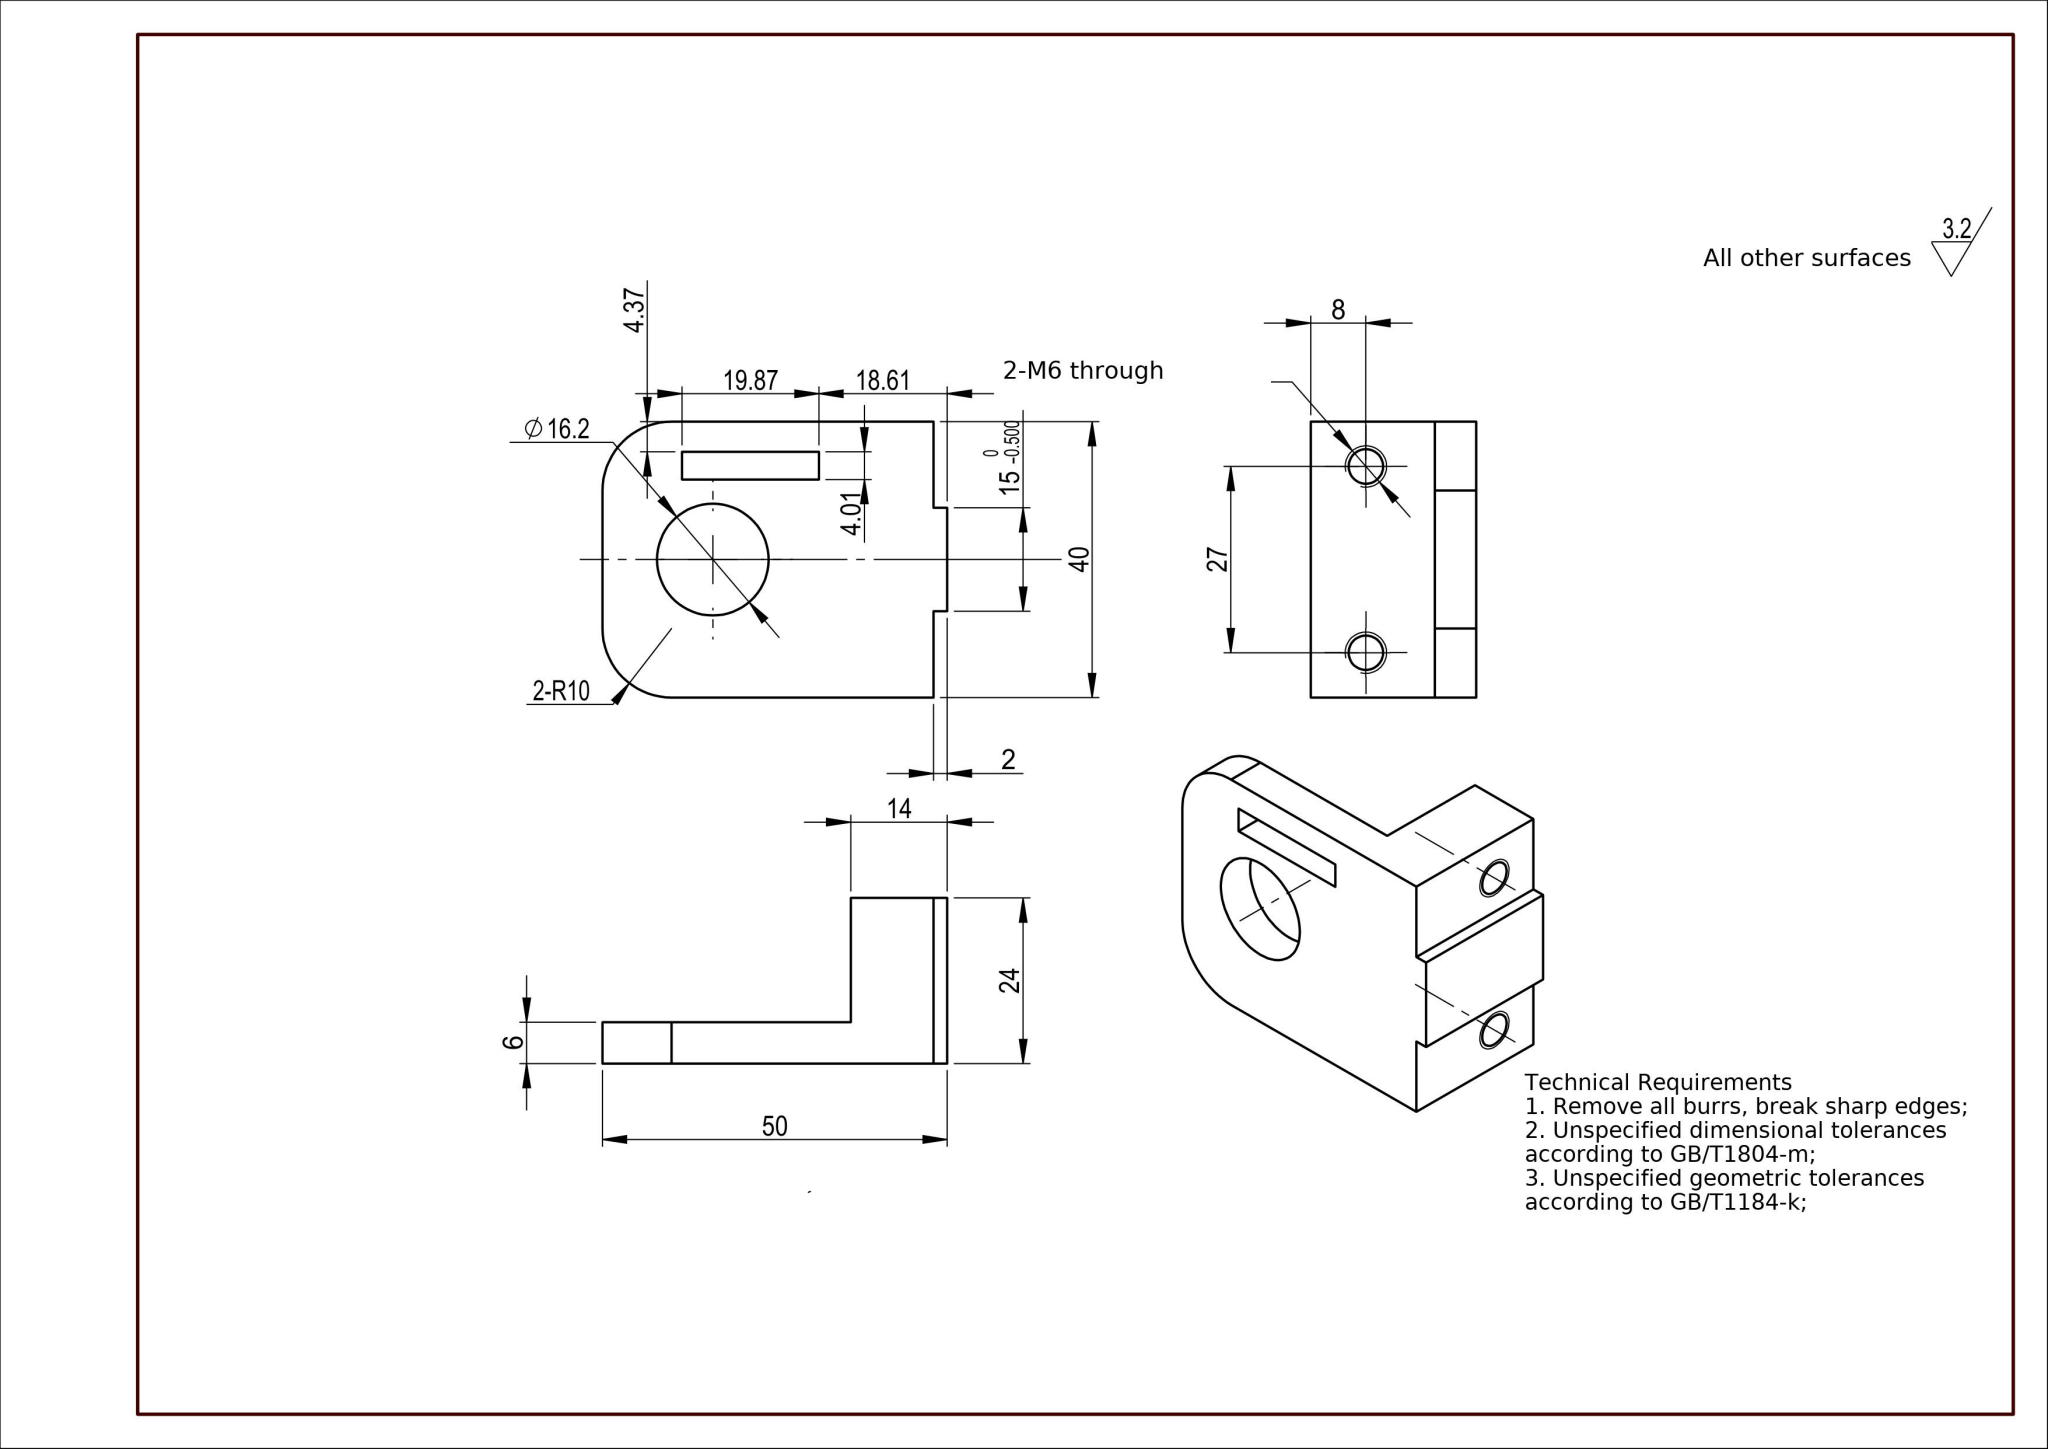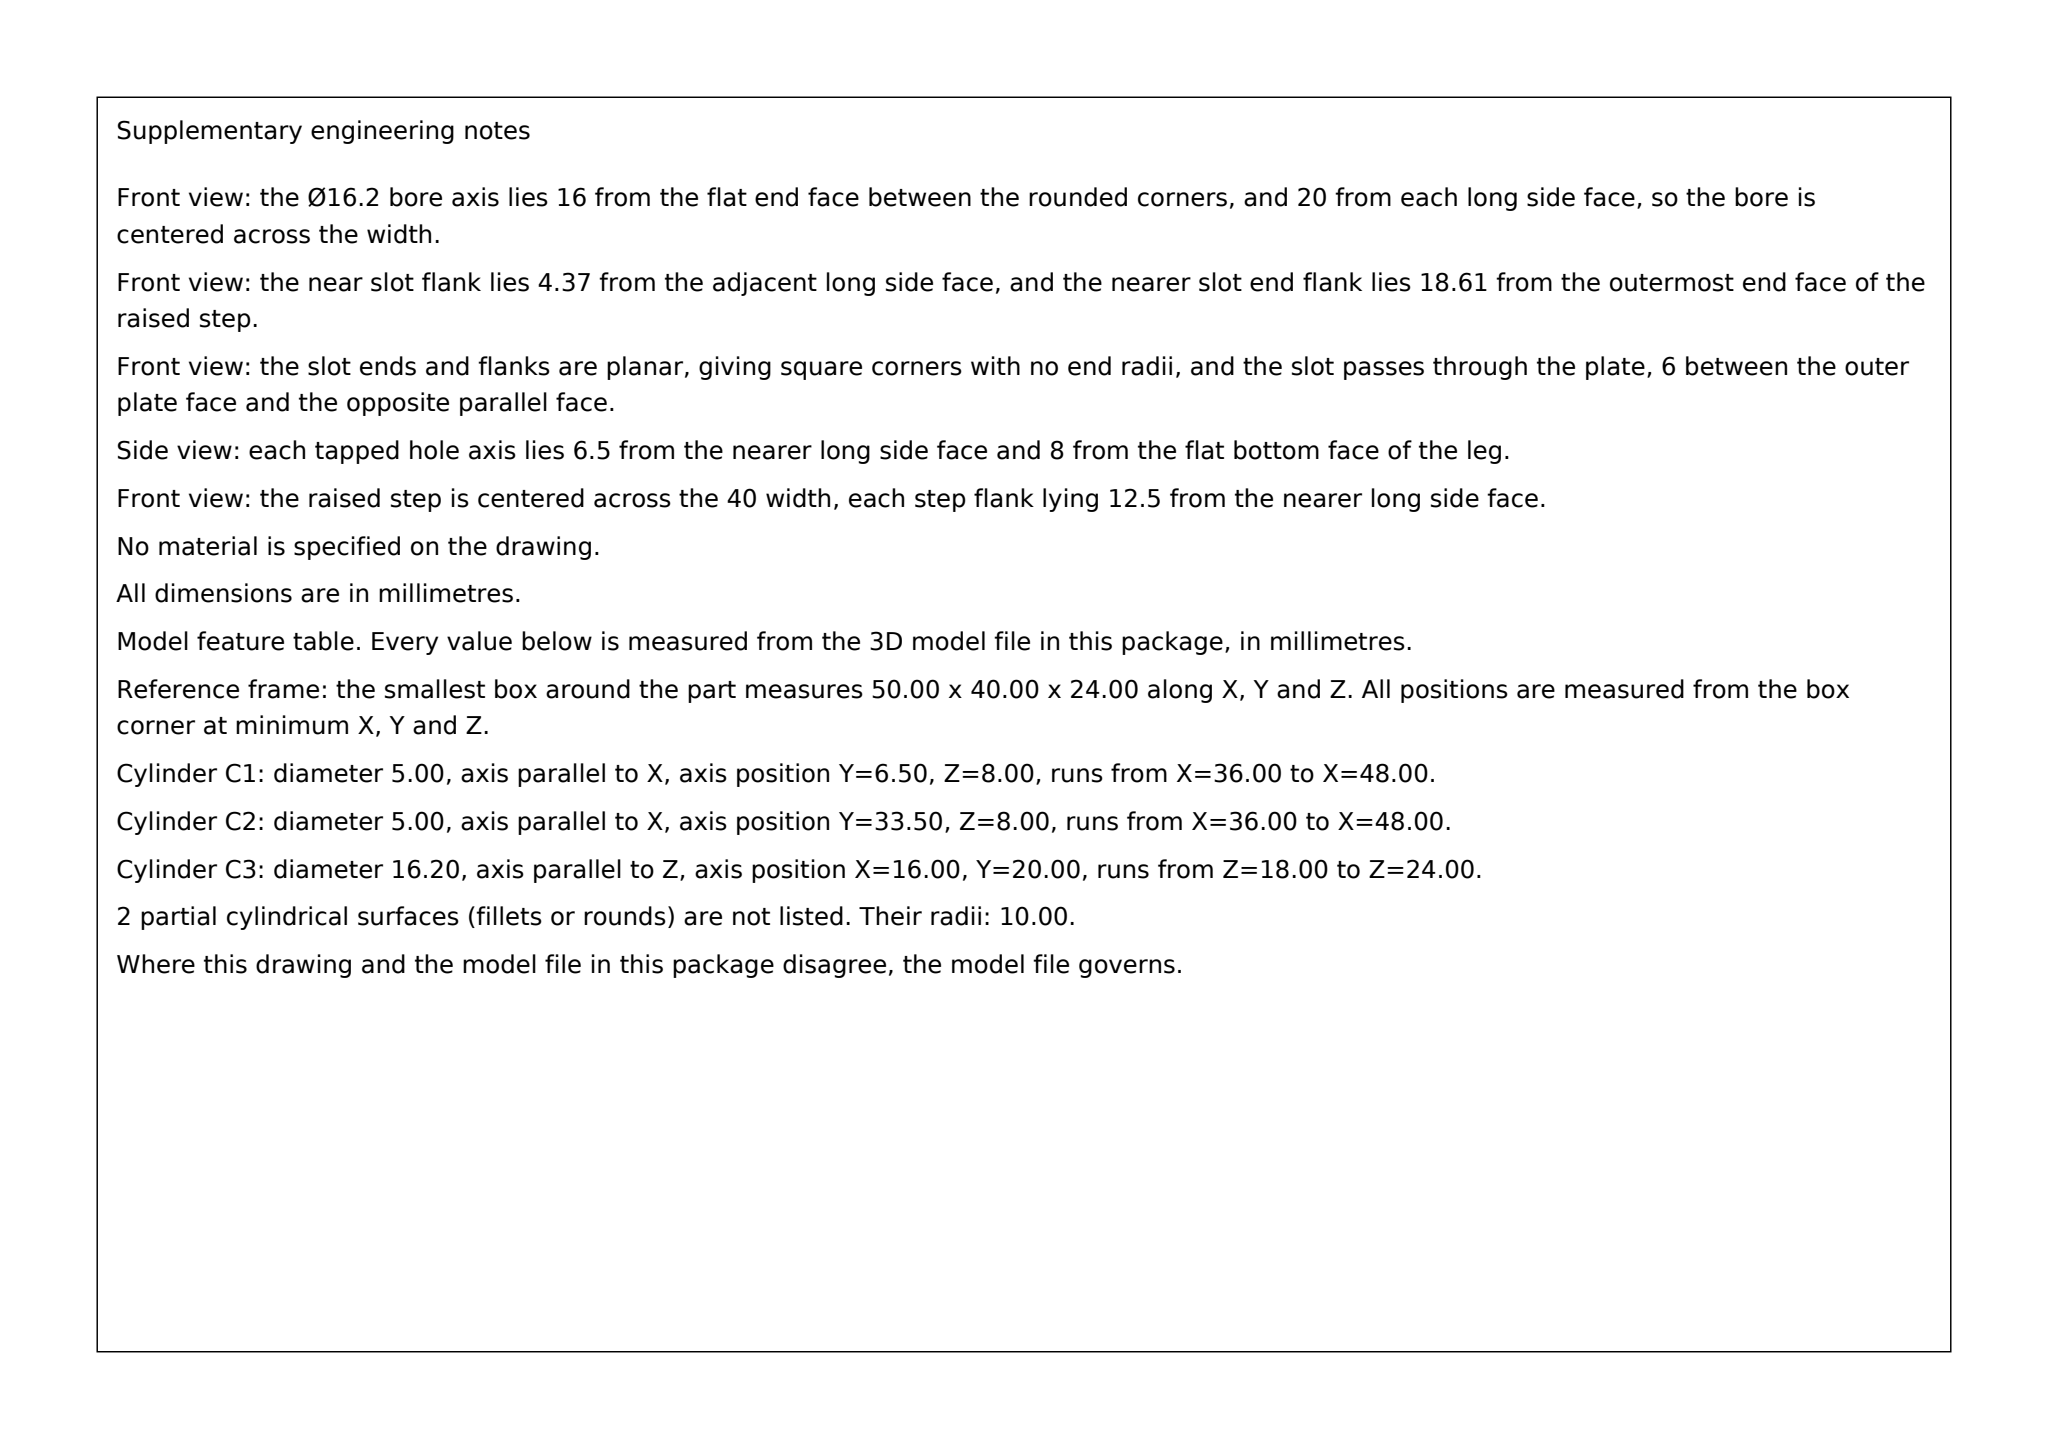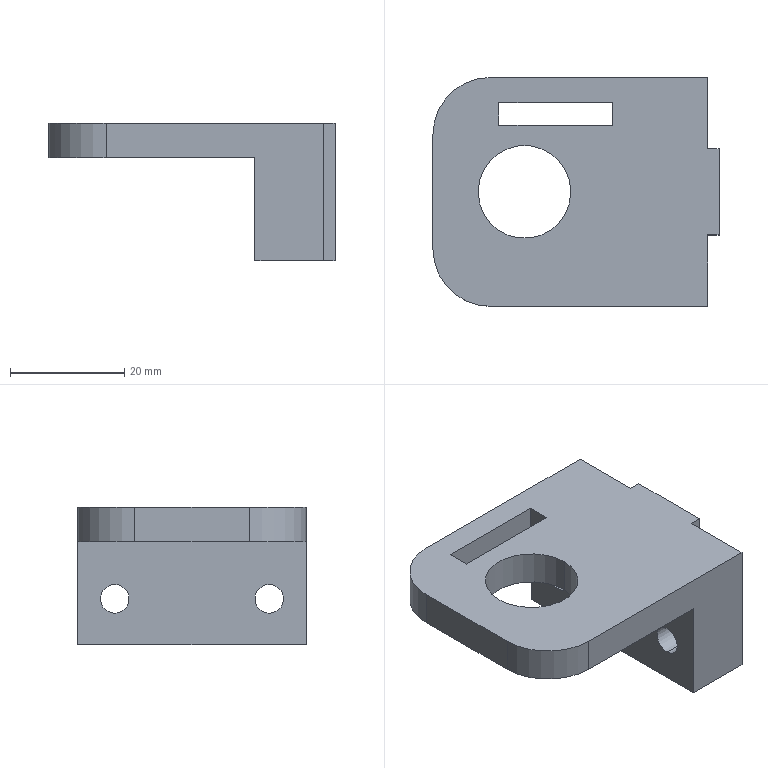Part | SolidWorks | mm | 1 solid | 24 faces | box 50 x 40 x 24 mm | volume 18436 mm3 | plane 16 | cylinder 8 | commonest cylinder face diameters 5 x4 16.2 x2 20 x2
Drawing notes:
PLAN VIEW: Ø16.2 HOLE CL 16 FROM LEFT FACE, ON 40 CL (20) | from the solid: cylinder dia 16.2, axis z, pos (x=16.0, y=20.0), bbox 50x40x24
PLAN VIEW: 19.87x4.01 SLOT LEFT END 11.52 FROM LEFT FACE | from the solid: x planes 11.52 & 31.39 (19.87 wide); y planes 31.61 & 35.63 (4.02 wide)
GROOVE 15 (0/-0.5) x 2 DP SYMM ABOUT 40 CL; 12.5 FROM EACH EDGE | from the solid: y-planes at 12.5 and 27.5 within 40 bbox width (15 wide, 12.5 each side)
SLOT 19.87 x 4.01 THRU 6 THK PLATE | from the solid: x-planes 11.52/31.39 = 19.87; y-planes 31.61/35.63 = 4.02; plate 6 thk (z 18-24, per Ø16.2 cyl length 6)
build123d program:
from build123d import *

# Parameters (mm, degrees)
SKETCH1_W             = 60
SKETCH1_H             = 40
BOSS_EXTRUDE1_DEPTH   = 3
SKETCH4_R             = 8.1
CUT_EXTRUDE1_DEPTH    = 37.551
FILLET1_R             = 10
CHAMFER1_SIZE         = 2
SKETCH6_W             = 12
SKETCH6_H             = 81.817
CUT_EXTRUDE2_DEPTH    = 10
SKETCH8_W             = 12
SKETCH8_H             = 40
BOSS_EXTRUDE2_DEPTH   = 18
M6_TAPPED_HOLE1_D     = 5
M6_TAPPED_HOLE1_DEPTH = 15
M6_TAPPED_HOLE1_TIP   = 1.502
SKETCH11_W            = 24
SKETCH11_H            = 15
BOSS_EXTRUDE3_DEPTH   = 2
SKETCH12_W            = 19.866
SKETCH12_H            = 4.014
CUT_EXTRUDE3_DEPTH    = 10


with BuildPart() as part:
    # Sketch1 → Boss-Extrude1 (new, symmetric)
    with BuildSketch(Plane.XY):
        Rectangle(SKETCH1_W, SKETCH1_H)
    extrude(amount=BOSS_EXTRUDE1_DEPTH, both=True)

    # Sketch4 → Cut-Extrude1 (cut, through all)
    with BuildSketch(Plane.XY.offset(3)):
        with Locations((-14, 0)):
            Circle(SKETCH4_R)
    extrude(amount=-CUT_EXTRUDE1_DEPTH, mode=Mode.SUBTRACT)

    # Fillet1
    fillet1_edges = [part.edges().sort_by_distance(p)[0] for p in [
        (-30, -20, 0),
        (-30, 20, 0),
    ]]
    fillet(fillet1_edges, radius=FILLET1_R)

    # Chamfer1
    chamfer1_edges = [part.edges().sort_by_distance(p)[0] for p in [
        (30, -20, 0),
        (30, 20, 0),
    ]]
    chamfer(chamfer1_edges, length=CHAMFER1_SIZE)

    # Sketch6 → Cut-Extrude2 (cut)
    with BuildSketch(Plane(origin=(0, 0, -3), x_dir=(-1, 0, 0), z_dir=(0, 0, -1))):
        with Locations((-24, -11.215)):
            Rectangle(SKETCH6_W, SKETCH6_H)
    extrude(amount=-CUT_EXTRUDE2_DEPTH, mode=Mode.SUBTRACT)

    # Sketch8 → Boss-Extrude2 (add)
    with BuildSketch(Plane(origin=(0, 0, -3), x_dir=(-1, 0, 0), z_dir=(0, 0, -1))):
        with Locations((-12, 0)):
            Rectangle(SKETCH8_W, SKETCH8_H)
    extrude(amount=BOSS_EXTRUDE2_DEPTH)

    # M6 Tapped Hole1
    with Locations(Plane(origin=(18, 0, 0), x_dir=(0, 0, -1), z_dir=(1, 0, 0))):
        with Locations((13, 13.5), (13, -13.5)):
            Hole(M6_TAPPED_HOLE1_D / 2, depth=M6_TAPPED_HOLE1_DEPTH)
            with Locations((0, 0, -(M6_TAPPED_HOLE1_DEPTH + M6_TAPPED_HOLE1_TIP / 2))):  # 118° drill point
                Cone(0, M6_TAPPED_HOLE1_D / 2, M6_TAPPED_HOLE1_TIP, mode=Mode.SUBTRACT)

    # Sketch11 → Boss-Extrude3 (add)
    with BuildSketch(Plane(origin=(18, 0, 0), x_dir=(0, 0, -1), z_dir=(1, 0, 0))):
        with Locations((9, 0)):
            Rectangle(SKETCH11_W, SKETCH11_H)
    extrude(amount=BOSS_EXTRUDE3_DEPTH)

    # Sketch12 → Cut-Extrude3 (cut)
    with BuildSketch(Plane(origin=(0, 0, -3), x_dir=(-1, 0, 0), z_dir=(0, 0, -1))):
        with Locations((8.543, 13.619)):
            Rectangle(SKETCH12_W, SKETCH12_H)
    extrude(amount=-CUT_EXTRUDE3_DEPTH, mode=Mode.SUBTRACT)


solid = part.part
STEP:
#1=CARTESIAN_POINT('',(6.,13.5,-10.5));
#2=VERTEX_POINT('',#1);
#3=CARTESIAN_POINT('',(6.,13.5,-15.5));
#4=VERTEX_POINT('',#3);
#5=CARTESIAN_POINT('',(6.,13.5,-13.));
#6=DIRECTION('',(1.,-0.,0.));
#7=DIRECTION('',(0.,1.,0.));
#8=AXIS2_PLACEMENT_3D('',#5,#6,#7);
#9=CIRCLE('',#8,2.5);
#10=EDGE_CURVE('',#2,#4,#9,.T.);
#11=ORIENTED_EDGE('',*,*,#10,.F.);
#12=CARTESIAN_POINT('',(18.,13.5,-10.5));
#13=VERTEX_POINT('',#12);
#14=CARTESIAN_POINT('',(18.,13.5,-10.5));
#15=DIRECTION('',(1.,0.,0.));
#16=VECTOR('',#15,1000.);
#17=LINE('',#14,#16);
#18=EDGE_CURVE('',#2,#13,#17,.T.);
#19=ORIENTED_EDGE('',*,*,#18,.T.);
#20=CARTESIAN_POINT('',(18.,13.5,-15.5));
#21=VERTEX_POINT('',#20);
#22=CARTESIAN_POINT('',(18.,13.5,-13.));
#23=DIRECTION('',(1.,0.,0.));
#24=DIRECTION('',(0.,0.,-1.));
#25=AXIS2_PLACEMENT_3D('',#22,#23,#24);
#26=CIRCLE('',#25,2.5);
#27=EDGE_CURVE('',#13,#21,#26,.T.);
#28=ORIENTED_EDGE('',*,*,#27,.T.);
#29=CARTESIAN_POINT('',(18.,13.5,-15.5));
#30=DIRECTION('',(1.,0.,0.));
#31=VECTOR('',#30,1000.);
#32=LINE('',#29,#31);
#33=EDGE_CURVE('',#4,#21,#32,.T.);
#34=ORIENTED_EDGE('',*,*,#33,.F.);
#35=EDGE_LOOP('',(#11,#19,#28,#34));
#36=FACE_OUTER_BOUND('',#35,.T.);
#37=CARTESIAN_POINT('',(18.,13.5,-13.));
#38=DIRECTION('',(1.,0.,0.));
#39=DIRECTION('',(0.,0.,-1.));
#40=AXIS2_PLACEMENT_3D('',#37,#38,#39);
#41=CYLINDRICAL_SURFACE('',#40,2.5);
#42=ADVANCED_FACE('',(#36),#41,.F.);
#43=CARTESIAN_POINT('',(6.,-13.5,-10.5));
#44=VERTEX_POINT('',#43);
#45=CARTESIAN_POINT('',(6.,-13.5,-15.5));
#46=VERTEX_POINT('',#45);
#47=CARTESIAN_POINT('',(6.,-13.5,-13.));
#48=DIRECTION('',(1.,-0.,0.));
#49=DIRECTION('',(0.,1.,0.));
#50=AXIS2_PLACEMENT_3D('',#47,#48,#49);
#51=CIRCLE('',#50,2.5);
#52=EDGE_CURVE('',#44,#46,#51,.T.);
#53=ORIENTED_EDGE('',*,*,#52,.F.);
#54=CARTESIAN_POINT('',(18.,-13.5,-10.5));
#55=VERTEX_POINT('',#54);
#56=CARTESIAN_POINT('',(18.,-13.5,-10.5));
#57=DIRECTION('',(1.,0.,0.));
#58=VECTOR('',#57,1000.);
#59=LINE('',#56,#58);
#60=EDGE_CURVE('',#44,#55,#59,.T.);
#61=ORIENTED_EDGE('',*,*,#60,.T.);
#62=CARTESIAN_POINT('',(18.,-13.5,-15.5));
#63=VERTEX_POINT('',#62);
#64=CARTESIAN_POINT('',(18.,-13.5,-13.));
#65=DIRECTION('',(1.,0.,0.));
#66=DIRECTION('',(0.,0.,-1.));
#67=AXIS2_PLACEMENT_3D('',#64,#65,#66);
#68=CIRCLE('',#67,2.5);
#69=EDGE_CURVE('',#55,#63,#68,.T.);
#70=ORIENTED_EDGE('',*,*,#69,.T.);
#71=CARTESIAN_POINT('',(18.,-13.5,-15.5));
#72=DIRECTION('',(1.,0.,0.));
#73=VECTOR('',#72,1000.);
#74=LINE('',#71,#73);
#75=EDGE_CURVE('',#46,#63,#74,.T.);
#76=ORIENTED_EDGE('',*,*,#75,.F.);
#77=EDGE_LOOP('',(#53,#61,#70,#76));
#78=FACE_OUTER_BOUND('',#77,.T.);
#79=CARTESIAN_POINT('',(18.,-13.5,-13.));
#80=DIRECTION('',(1.,0.,0.));
#81=DIRECTION('',(0.,0.,-1.));
#82=AXIS2_PLACEMENT_3D('',#79,#80,#81);
#83=CYLINDRICAL_SURFACE('',#82,2.5);
#84=ADVANCED_FACE('',(#78),#83,.F.);
#85=CARTESIAN_POINT('',(-22.1,0.,-3.));
#86=VERTEX_POINT('',#85);
#87=CARTESIAN_POINT('',(-5.9,0.,-3.));
#88=VERTEX_POINT('',#87);
#89=CARTESIAN_POINT('',(-14.,0.,-3.));
#90=DIRECTION('',(0.,0.,1.));
#91=DIRECTION('',(1.,0.,0.));
#92=AXIS2_PLACEMENT_3D('',#89,#90,#91);
#93=CIRCLE('',#92,8.1);
#94=EDGE_CURVE('',#86,#88,#93,.T.);
#95=ORIENTED_EDGE('',*,*,#94,.F.);
#96=CARTESIAN_POINT('',(-22.1,0.,3.));
#97=VERTEX_POINT('',#96);
#98=CARTESIAN_POINT('',(-22.1,0.,-3.));
#99=DIRECTION('',(0.,0.,1.));
#100=VECTOR('',#99,1000.);
#101=LINE('',#98,#100);
#102=EDGE_CURVE('',#86,#97,#101,.T.);
#103=ORIENTED_EDGE('',*,*,#102,.T.);
#104=CARTESIAN_POINT('',(-5.9,0.,3.));
#105=VERTEX_POINT('',#104);
#106=CARTESIAN_POINT('',(-14.,0.,3.));
#107=DIRECTION('',(0.,0.,1.));
#108=DIRECTION('',(1.,0.,0.));
#109=AXIS2_PLACEMENT_3D('',#106,#107,#108);
#110=CIRCLE('',#109,8.1);
#111=EDGE_CURVE('',#97,#105,#110,.T.);
#112=ORIENTED_EDGE('',*,*,#111,.T.);
#113=CARTESIAN_POINT('',(-5.9,0.,-3.));
#114=DIRECTION('',(0.,0.,1.));
#115=VECTOR('',#114,1000.);
#116=LINE('',#113,#115);
#117=EDGE_CURVE('',#88,#105,#116,.T.);
#118=ORIENTED_EDGE('',*,*,#117,.F.);
#119=EDGE_LOOP('',(#95,#103,#112,#118));
#120=FACE_OUTER_BOUND('',#119,.T.);
#121=CARTESIAN_POINT('',(-14.,0.,-3.));
#122=DIRECTION('',(0.,0.,1.));
#123=DIRECTION('',(1.,0.,0.));
#124=AXIS2_PLACEMENT_3D('',#121,#122,#123);
#125=CYLINDRICAL_SURFACE('',#124,8.1);
#126=ADVANCED_FACE('',(#120),#125,.F.);
#127=CARTESIAN_POINT('',(18.,-13.5,-13.));
#128=DIRECTION('',(1.,0.,0.));
#129=DIRECTION('',(0.,0.,-1.));
#130=AXIS2_PLACEMENT_3D('',#127,#128,#129);
#131=CIRCLE('',#130,2.5);
#132=EDGE_CURVE('',#63,#55,#131,.T.);
#133=ORIENTED_EDGE('',*,*,#132,.F.);
#134=ORIENTED_EDGE('',*,*,#69,.F.);
#135=EDGE_LOOP('',(#133,#134));
#136=FACE_BOUND('',#135,.T.);
#137=CARTESIAN_POINT('',(18.,-7.5,3.));
#138=VERTEX_POINT('',#137);
#139=CARTESIAN_POINT('',(18.,-7.5,-21.));
#140=VERTEX_POINT('',#139);
#141=CARTESIAN_POINT('',(18.,-7.5,3.));
#142=DIRECTION('',(0.,0.,-1.));
#143=VECTOR('',#142,1000.);
#144=LINE('',#141,#143);
#145=EDGE_CURVE('',#138,#140,#144,.T.);
#146=ORIENTED_EDGE('',*,*,#145,.F.);
#147=CARTESIAN_POINT('',(18.,-20.,3.));
#148=VERTEX_POINT('',#147);
#149=CARTESIAN_POINT('',(18.,20.,3.));
#150=DIRECTION('',(0.,1.,0.));
#151=VECTOR('',#150,1000.);
#152=LINE('',#149,#151);
#153=EDGE_CURVE('',#148,#138,#152,.T.);
#154=ORIENTED_EDGE('',*,*,#153,.F.);
#155=CARTESIAN_POINT('',(18.,-20.,-21.));
#156=VERTEX_POINT('',#155);
#157=CARTESIAN_POINT('',(18.,-20.,3.));
#158=DIRECTION('',(0.,0.,1.));
#159=VECTOR('',#158,1000.);
#160=LINE('',#157,#159);
#161=EDGE_CURVE('',#156,#148,#160,.T.);
#162=ORIENTED_EDGE('',*,*,#161,.F.);
#163=CARTESIAN_POINT('',(18.,20.,-21.));
#164=DIRECTION('',(0.,-1.,0.));
#165=VECTOR('',#164,1000.);
#166=LINE('',#163,#165);
#167=EDGE_CURVE('',#140,#156,#166,.T.);
#168=ORIENTED_EDGE('',*,*,#167,.F.);
#169=EDGE_LOOP('',(#146,#154,#162,#168));
#170=FACE_OUTER_BOUND('',#169,.T.);
#171=CARTESIAN_POINT('',(18.,-52.123,7.));
#172=DIRECTION('',(-1.,0.,0.));
#173=DIRECTION('',(0.,0.,1.));
#174=AXIS2_PLACEMENT_3D('',#171,#172,#173);
#175=PLANE('',#174);
#176=ADVANCED_FACE('',(#136,#170),#175,.F.);
#177=CARTESIAN_POINT('',(18.,13.5,-13.));
#178=DIRECTION('',(1.,0.,0.));
#179=DIRECTION('',(0.,0.,-1.));
#180=AXIS2_PLACEMENT_3D('',#177,#178,#179);
#181=CIRCLE('',#180,2.5);
#182=EDGE_CURVE('',#21,#13,#181,.T.);
#183=ORIENTED_EDGE('',*,*,#182,.F.);
#184=ORIENTED_EDGE('',*,*,#27,.F.);
#185=EDGE_LOOP('',(#183,#184));
#186=FACE_BOUND('',#185,.T.);
#187=CARTESIAN_POINT('',(18.,7.5,-21.));
#188=VERTEX_POINT('',#187);
#189=CARTESIAN_POINT('',(18.,7.5,3.));
#190=VERTEX_POINT('',#189);
#191=CARTESIAN_POINT('',(18.,7.5,3.));
#192=DIRECTION('',(0.,0.,1.));
#193=VECTOR('',#192,1000.);
#194=LINE('',#191,#193);
#195=EDGE_CURVE('',#188,#190,#194,.T.);
#196=ORIENTED_EDGE('',*,*,#195,.F.);
#197=CARTESIAN_POINT('',(18.,20.,-21.));
#198=VERTEX_POINT('',#197);
#199=CARTESIAN_POINT('',(18.,20.,-21.));
#200=DIRECTION('',(0.,-1.,0.));
#201=VECTOR('',#200,1000.);
#202=LINE('',#199,#201);
#203=EDGE_CURVE('',#198,#188,#202,.T.);
#204=ORIENTED_EDGE('',*,*,#203,.F.);
#205=CARTESIAN_POINT('',(18.,20.,3.));
#206=VERTEX_POINT('',#205);
#207=CARTESIAN_POINT('',(18.,20.,3.));
#208=DIRECTION('',(0.,0.,-1.));
#209=VECTOR('',#208,1000.);
#210=LINE('',#207,#209);
#211=EDGE_CURVE('',#206,#198,#210,.T.);
#212=ORIENTED_EDGE('',*,*,#211,.F.);
#213=CARTESIAN_POINT('',(18.,20.,3.));
#214=DIRECTION('',(0.,1.,0.));
#215=VECTOR('',#214,1000.);
#216=LINE('',#213,#215);
#217=EDGE_CURVE('',#190,#206,#216,.T.);
#218=ORIENTED_EDGE('',*,*,#217,.F.);
#219=EDGE_LOOP('',(#196,#204,#212,#218));
#220=FACE_OUTER_BOUND('',#219,.T.);
#221=CARTESIAN_POINT('',(18.,-52.123,7.));
#222=DIRECTION('',(-1.,0.,0.));
#223=DIRECTION('',(0.,0.,1.));
#224=AXIS2_PLACEMENT_3D('',#221,#222,#223);
#225=PLANE('',#224);
#226=ADVANCED_FACE('',(#186,#220),#225,.F.);
#227=CARTESIAN_POINT('',(-20.,20.,3.));
#228=VERTEX_POINT('',#227);
#229=CARTESIAN_POINT('',(-30.,20.,3.));
#230=DIRECTION('',(-1.,0.,0.));
#231=VECTOR('',#230,1000.);
#232=LINE('',#229,#231);
#233=EDGE_CURVE('',#206,#228,#232,.T.);
#234=ORIENTED_EDGE('',*,*,#233,.F.);
#235=ORIENTED_EDGE('',*,*,#211,.T.);
#236=CARTESIAN_POINT('',(6.,20.,-21.));
#237=VERTEX_POINT('',#236);
#238=CARTESIAN_POINT('',(6.,20.,-21.));
#239=DIRECTION('',(1.,-0.,0.));
#240=VECTOR('',#239,1000.);
#241=LINE('',#238,#240);
#242=EDGE_CURVE('',#237,#198,#241,.T.);
#243=ORIENTED_EDGE('',*,*,#242,.F.);
#244=CARTESIAN_POINT('',(6.,20.,-3.));
#245=VERTEX_POINT('',#244);
#246=CARTESIAN_POINT('',(6.,20.,-21.));
#247=DIRECTION('',(0.,0.,1.));
#248=VECTOR('',#247,1000.);
#249=LINE('',#246,#248);
#250=EDGE_CURVE('',#237,#245,#249,.T.);
#251=ORIENTED_EDGE('',*,*,#250,.T.);
#252=CARTESIAN_POINT('',(-20.,20.,-3.));
#253=VERTEX_POINT('',#252);
#254=CARTESIAN_POINT('',(-30.,20.,-3.));
#255=DIRECTION('',(-1.,0.,0.));
#256=VECTOR('',#255,1000.);
#257=LINE('',#254,#256);
#258=EDGE_CURVE('',#245,#253,#257,.T.);
#259=ORIENTED_EDGE('',*,*,#258,.T.);
#260=CARTESIAN_POINT('',(-20.,20.,3.));
#261=DIRECTION('',(0.,0.,1.));
#262=VECTOR('',#261,1000.);
#263=LINE('',#260,#262);
#264=EDGE_CURVE('',#253,#228,#263,.T.);
#265=ORIENTED_EDGE('',*,*,#264,.T.);
#266=EDGE_LOOP('',(#234,#235,#243,#251,#259,#265));
#267=FACE_OUTER_BOUND('',#266,.T.);
#268=CARTESIAN_POINT('',(-30.,20.,3.));
#269=DIRECTION('',(0.,-1.,0.));
#270=DIRECTION('',(0.,0.,-1.));
#271=AXIS2_PLACEMENT_3D('',#268,#269,#270);
#272=PLANE('',#271);
#273=ADVANCED_FACE('',(#267),#272,.F.);
#274=CARTESIAN_POINT('',(-30.,10.,-3.));
#275=VERTEX_POINT('',#274);
#276=CARTESIAN_POINT('',(-30.,-10.,-3.));
#277=VERTEX_POINT('',#276);
#278=CARTESIAN_POINT('',(-30.,-20.,-3.));
#279=DIRECTION('',(0.,-1.,0.));
#280=VECTOR('',#279,1000.);
#281=LINE('',#278,#280);
#282=EDGE_CURVE('',#275,#277,#281,.T.);
#283=ORIENTED_EDGE('',*,*,#282,.T.);
#284=CARTESIAN_POINT('',(-30.,-10.,3.));
#285=VERTEX_POINT('',#284);
#286=CARTESIAN_POINT('',(-30.,-10.,3.));
#287=DIRECTION('',(0.,0.,1.));
#288=VECTOR('',#287,1000.);
#289=LINE('',#286,#288);
#290=EDGE_CURVE('',#277,#285,#289,.T.);
#291=ORIENTED_EDGE('',*,*,#290,.T.);
#292=CARTESIAN_POINT('',(-30.,10.,3.));
#293=VERTEX_POINT('',#292);
#294=CARTESIAN_POINT('',(-30.,-20.,3.));
#295=DIRECTION('',(0.,-1.,0.));
#296=VECTOR('',#295,1000.);
#297=LINE('',#294,#296);
#298=EDGE_CURVE('',#293,#285,#297,.T.);
#299=ORIENTED_EDGE('',*,*,#298,.F.);
#300=CARTESIAN_POINT('',(-30.,10.,3.));
#301=DIRECTION('',(0.,0.,-1.));
#302=VECTOR('',#301,1000.);
#303=LINE('',#300,#302);
#304=EDGE_CURVE('',#293,#275,#303,.T.);
#305=ORIENTED_EDGE('',*,*,#304,.T.);
#306=EDGE_LOOP('',(#283,#291,#299,#305));
#307=FACE_OUTER_BOUND('',#306,.T.);
#308=CARTESIAN_POINT('',(-30.,-20.,3.));
#309=DIRECTION('',(1.,0.,0.));
#310=DIRECTION('',(0.,0.,-1.));
#311=AXIS2_PLACEMENT_3D('',#308,#309,#310);
#312=PLANE('',#311);
#313=ADVANCED_FACE('',(#307),#312,.F.);
#314=CARTESIAN_POINT('',(-20.,-20.,-3.));
#315=VERTEX_POINT('',#314);
#316=CARTESIAN_POINT('',(6.,-20.,-3.));
#317=VERTEX_POINT('',#316);
#318=CARTESIAN_POINT('',(-30.,-20.,-3.));
#319=DIRECTION('',(1.,0.,0.));
#320=VECTOR('',#319,1000.);
#321=LINE('',#318,#320);
#322=EDGE_CURVE('',#315,#317,#321,.T.);
#323=ORIENTED_EDGE('',*,*,#322,.T.);
#324=CARTESIAN_POINT('',(6.,-20.,-21.));
#325=VERTEX_POINT('',#324);
#326=CARTESIAN_POINT('',(6.,-20.,-21.));
#327=DIRECTION('',(0.,0.,1.));
#328=VECTOR('',#327,1000.);
#329=LINE('',#326,#328);
#330=EDGE_CURVE('',#325,#317,#329,.T.);
#331=ORIENTED_EDGE('',*,*,#330,.F.);
#332=CARTESIAN_POINT('',(6.,-20.,-21.));
#333=DIRECTION('',(-1.,0.,0.));
#334=VECTOR('',#333,1000.);
#335=LINE('',#332,#334);
#336=EDGE_CURVE('',#156,#325,#335,.T.);
#337=ORIENTED_EDGE('',*,*,#336,.F.);
#338=ORIENTED_EDGE('',*,*,#161,.T.);
#339=CARTESIAN_POINT('',(-20.,-20.,3.));
#340=VERTEX_POINT('',#339);
#341=CARTESIAN_POINT('',(-30.,-20.,3.));
#342=DIRECTION('',(1.,0.,0.));
#343=VECTOR('',#342,1000.);
#344=LINE('',#341,#343);
#345=EDGE_CURVE('',#340,#148,#344,.T.);
#346=ORIENTED_EDGE('',*,*,#345,.F.);
#347=CARTESIAN_POINT('',(-20.,-20.,3.));
#348=DIRECTION('',(0.,0.,-1.));
#349=VECTOR('',#348,1000.);
#350=LINE('',#347,#349);
#351=EDGE_CURVE('',#340,#315,#350,.T.);
#352=ORIENTED_EDGE('',*,*,#351,.T.);
#353=EDGE_LOOP('',(#323,#331,#337,#338,#346,#352));
#354=FACE_OUTER_BOUND('',#353,.T.);
#355=CARTESIAN_POINT('',(-30.,-20.,3.));
#356=DIRECTION('',(0.,1.,0.));
#357=DIRECTION('',(0.,0.,1.));
#358=AXIS2_PLACEMENT_3D('',#355,#356,#357);
#359=PLANE('',#358);
#360=ADVANCED_FACE('',(#354),#359,.F.);
#361=CARTESIAN_POINT('',(-18.476,15.626,3.));
#362=VERTEX_POINT('',#361);
#363=CARTESIAN_POINT('',(1.39,15.626,3.));
#364=VERTEX_POINT('',#363);
#365=CARTESIAN_POINT('',(30.,15.626,3.));
#366=DIRECTION('',(1.,0.,0.));
#367=VECTOR('',#366,1000.);
#368=LINE('',#365,#367);
#369=EDGE_CURVE('',#362,#364,#368,.T.);
#370=ORIENTED_EDGE('',*,*,#369,.T.);
#371=CARTESIAN_POINT('',(1.39,11.612,3.));
#372=VERTEX_POINT('',#371);
#373=CARTESIAN_POINT('',(1.39,20.,3.));
#374=DIRECTION('',(0.,-1.,0.));
#375=VECTOR('',#374,1000.);
#376=LINE('',#373,#375);
#377=EDGE_CURVE('',#364,#372,#376,.T.);
#378=ORIENTED_EDGE('',*,*,#377,.T.);
#379=CARTESIAN_POINT('',(-18.476,11.612,3.));
#380=VERTEX_POINT('',#379);
#381=CARTESIAN_POINT('',(30.,11.612,3.));
#382=DIRECTION('',(-1.,0.,0.));
#383=VECTOR('',#382,1000.);
#384=LINE('',#381,#383);
#385=EDGE_CURVE('',#372,#380,#384,.T.);
#386=ORIENTED_EDGE('',*,*,#385,.T.);
#387=CARTESIAN_POINT('',(-18.476,20.,3.));
#388=DIRECTION('',(0.,1.,0.));
#389=VECTOR('',#388,1000.);
#390=LINE('',#387,#389);
#391=EDGE_CURVE('',#380,#362,#390,.T.);
#392=ORIENTED_EDGE('',*,*,#391,.T.);
#393=EDGE_LOOP('',(#370,#378,#386,#392));
#394=FACE_BOUND('',#393,.T.);
#395=CARTESIAN_POINT('',(-14.,0.,3.));
#396=DIRECTION('',(0.,0.,1.));
#397=DIRECTION('',(1.,0.,0.));
#398=AXIS2_PLACEMENT_3D('',#395,#396,#397);
#399=CIRCLE('',#398,8.1);
#400=EDGE_CURVE('',#105,#97,#399,.T.);
#401=ORIENTED_EDGE('',*,*,#400,.F.);
#402=ORIENTED_EDGE('',*,*,#111,.F.);
#403=EDGE_LOOP('',(#401,#402));
#404=FACE_BOUND('',#403,.T.);
#405=ORIENTED_EDGE('',*,*,#345,.T.);
#406=ORIENTED_EDGE('',*,*,#153,.T.);
#407=CARTESIAN_POINT('',(20.,-7.5,3.));
#408=VERTEX_POINT('',#407);
#409=CARTESIAN_POINT('',(20.,-7.5,3.));
#410=DIRECTION('',(-1.,0.,0.));
#411=VECTOR('',#410,1000.);
#412=LINE('',#409,#411);
#413=EDGE_CURVE('',#408,#138,#412,.T.);
#414=ORIENTED_EDGE('',*,*,#413,.F.);
#415=CARTESIAN_POINT('',(20.,7.5,3.));
#416=VERTEX_POINT('',#415);
#417=CARTESIAN_POINT('',(20.,7.5,3.));
#418=DIRECTION('',(0.,-1.,-0.));
#419=VECTOR('',#418,1000.);
#420=LINE('',#417,#419);
#421=EDGE_CURVE('',#416,#408,#420,.T.);
#422=ORIENTED_EDGE('',*,*,#421,.F.);
#423=CARTESIAN_POINT('',(20.,7.5,3.));
#424=DIRECTION('',(-1.,0.,0.));
#425=VECTOR('',#424,1000.);
#426=LINE('',#423,#425);
#427=EDGE_CURVE('',#416,#190,#426,.T.);
#428=ORIENTED_EDGE('',*,*,#427,.T.);
#429=ORIENTED_EDGE('',*,*,#217,.T.);
#430=ORIENTED_EDGE('',*,*,#233,.T.);
#431=CARTESIAN_POINT('',(-20.,10.,3.));
#432=DIRECTION('',(0.,0.,1.));
#433=DIRECTION('',(-1.,0.,0.));
#434=AXIS2_PLACEMENT_3D('',#431,#432,#433);
#435=CIRCLE('',#434,10.);
#436=EDGE_CURVE('',#228,#293,#435,.T.);
#437=ORIENTED_EDGE('',*,*,#436,.T.);
#438=ORIENTED_EDGE('',*,*,#298,.T.);
#439=CARTESIAN_POINT('',(-20.,-10.,3.));
#440=DIRECTION('',(0.,0.,1.));
#441=DIRECTION('',(-1.,0.,0.));
#442=AXIS2_PLACEMENT_3D('',#439,#440,#441);
#443=CIRCLE('',#442,10.);
#444=EDGE_CURVE('',#285,#340,#443,.T.);
#445=ORIENTED_EDGE('',*,*,#444,.T.);
#446=EDGE_LOOP('',(#405,#406,#414,#422,#428,#429,#430,#437,#438,#445));
#447=FACE_OUTER_BOUND('',#446,.T.);
#448=CARTESIAN_POINT('',(30.,20.,3.));
#449=DIRECTION('',(0.,0.,-1.));
#450=DIRECTION('',(-1.,0.,0.));
#451=AXIS2_PLACEMENT_3D('',#448,#449,#450);
#452=PLANE('',#451);
#453=ADVANCED_FACE('',(#394,#404,#447),#452,.F.);
#454=CARTESIAN_POINT('',(1.39,15.626,-3.));
#455=VERTEX_POINT('',#454);
#456=CARTESIAN_POINT('',(1.39,11.612,-3.));
#457=VERTEX_POINT('',#456);
#458=CARTESIAN_POINT('',(1.39,15.626,-3.));
#459=DIRECTION('',(0.,-1.,0.));
#460=VECTOR('',#459,1000.);
#461=LINE('',#458,#460);
#462=EDGE_CURVE('',#455,#457,#461,.T.);
#463=ORIENTED_EDGE('',*,*,#462,.F.);
#464=CARTESIAN_POINT('',(-18.476,15.626,-3.));
#465=VERTEX_POINT('',#464);
#466=CARTESIAN_POINT('',(1.39,15.626,-3.));
#467=DIRECTION('',(1.,0.,0.));
#468=VECTOR('',#467,1000.);
#469=LINE('',#466,#468);
#470=EDGE_CURVE('',#465,#455,#469,.T.);
#471=ORIENTED_EDGE('',*,*,#470,.F.);
#472=CARTESIAN_POINT('',(-18.476,11.612,-3.));
#473=VERTEX_POINT('',#472);
#474=CARTESIAN_POINT('',(-18.476,15.626,-3.));
#475=DIRECTION('',(0.,1.,0.));
#476=VECTOR('',#475,1000.);
#477=LINE('',#474,#476);
#478=EDGE_CURVE('',#473,#465,#477,.T.);
#479=ORIENTED_EDGE('',*,*,#478,.F.);
#480=CARTESIAN_POINT('',(1.39,11.612,-3.));
#481=DIRECTION('',(-1.,0.,0.));
#482=VECTOR('',#481,1000.);
#483=LINE('',#480,#482);
#484=EDGE_CURVE('',#457,#473,#483,.T.);
#485=ORIENTED_EDGE('',*,*,#484,.F.);
#486=EDGE_LOOP('',(#463,#471,#479,#485));
#487=FACE_BOUND('',#486,.T.);
#488=CARTESIAN_POINT('',(6.,20.,-3.));
#489=DIRECTION('',(0.,1.,0.));
#490=VECTOR('',#489,1000.);
#491=LINE('',#488,#490);
#492=EDGE_CURVE('',#317,#245,#491,.T.);
#493=ORIENTED_EDGE('',*,*,#492,.F.);
#494=ORIENTED_EDGE('',*,*,#322,.F.);
#495=CARTESIAN_POINT('',(-20.,-10.,-3.));
#496=DIRECTION('',(0.,0.,-1.));
#497=DIRECTION('',(-1.,0.,0.));
#498=AXIS2_PLACEMENT_3D('',#495,#496,#497);
#499=CIRCLE('',#498,10.);
#500=EDGE_CURVE('',#315,#277,#499,.T.);
#501=ORIENTED_EDGE('',*,*,#500,.T.);
#502=ORIENTED_EDGE('',*,*,#282,.F.);
#503=CARTESIAN_POINT('',(-20.,10.,-3.));
#504=DIRECTION('',(0.,0.,-1.));
#505=DIRECTION('',(-1.,0.,0.));
#506=AXIS2_PLACEMENT_3D('',#503,#504,#505);
#507=CIRCLE('',#506,10.);
#508=EDGE_CURVE('',#275,#253,#507,.T.);
#509=ORIENTED_EDGE('',*,*,#508,.T.);
#510=ORIENTED_EDGE('',*,*,#258,.F.);
#511=EDGE_LOOP('',(#493,#494,#501,#502,#509,#510));
#512=FACE_OUTER_BOUND('',#511,.T.);
#513=CARTESIAN_POINT('',(-14.,0.,-3.));
#514=DIRECTION('',(0.,0.,1.));
#515=DIRECTION('',(1.,0.,0.));
#516=AXIS2_PLACEMENT_3D('',#513,#514,#515);
#517=CIRCLE('',#516,8.1);
#518=EDGE_CURVE('',#88,#86,#517,.T.);
#519=ORIENTED_EDGE('',*,*,#518,.T.);
#520=ORIENTED_EDGE('',*,*,#94,.T.);
#521=EDGE_LOOP('',(#519,#520));
#522=FACE_BOUND('',#521,.T.);
#523=CARTESIAN_POINT('',(30.,20.,-3.));
#524=DIRECTION('',(0.,0.,-1.));
#525=DIRECTION('',(-1.,0.,0.));
#526=AXIS2_PLACEMENT_3D('',#523,#524,#525);
#527=PLANE('',#526);
#528=ADVANCED_FACE('',(#487,#512,#522),#527,.T.);
#529=ORIENTED_EDGE('',*,*,#102,.F.);
#530=ORIENTED_EDGE('',*,*,#518,.F.);
#531=ORIENTED_EDGE('',*,*,#117,.T.);
#532=ORIENTED_EDGE('',*,*,#400,.T.);
#533=EDGE_LOOP('',(#529,#530,#531,#532));
#534=FACE_OUTER_BOUND('',#533,.T.);
#535=CARTESIAN_POINT('',(-14.,0.,-3.));
#536=DIRECTION('',(0.,0.,1.));
#537=DIRECTION('',(1.,0.,0.));
#538=AXIS2_PLACEMENT_3D('',#535,#536,#537);
#539=CYLINDRICAL_SURFACE('',#538,8.1);
#540=ADVANCED_FACE('',(#534),#539,.F.);
#541=ORIENTED_EDGE('',*,*,#444,.F.);
#542=ORIENTED_EDGE('',*,*,#290,.F.);
#543=ORIENTED_EDGE('',*,*,#500,.F.);
#544=ORIENTED_EDGE('',*,*,#351,.F.);
#545=EDGE_LOOP('',(#541,#542,#543,#544));
#546=FACE_OUTER_BOUND('',#545,.T.);
#547=CARTESIAN_POINT('',(-20.,-10.,3.));
#548=DIRECTION('',(0.,0.,-1.));
#549=DIRECTION('',(-1.,0.,0.));
#550=AXIS2_PLACEMENT_3D('',#547,#548,#549);
#551=CYLINDRICAL_SURFACE('',#550,10.);
#552=ADVANCED_FACE('',(#546),#551,.T.);
#553=ORIENTED_EDGE('',*,*,#436,.F.);
#554=ORIENTED_EDGE('',*,*,#264,.F.);
#555=ORIENTED_EDGE('',*,*,#508,.F.);
#556=ORIENTED_EDGE('',*,*,#304,.F.);
#557=EDGE_LOOP('',(#553,#554,#555,#556));
#558=FACE_OUTER_BOUND('',#557,.T.);
#559=CARTESIAN_POINT('',(-20.,10.,3.));
#560=DIRECTION('',(0.,0.,-1.));
#561=DIRECTION('',(-1.,0.,0.));
#562=AXIS2_PLACEMENT_3D('',#559,#560,#561);
#563=CYLINDRICAL_SURFACE('',#562,10.);
#564=ADVANCED_FACE('',(#558),#563,.T.);
#565=CARTESIAN_POINT('',(6.,13.5,-13.));
#566=DIRECTION('',(1.,-0.,0.));
#567=DIRECTION('',(0.,1.,0.));
#568=AXIS2_PLACEMENT_3D('',#565,#566,#567);
#569=CIRCLE('',#568,2.5);
#570=EDGE_CURVE('',#4,#2,#569,.T.);
#571=ORIENTED_EDGE('',*,*,#570,.T.);
#572=ORIENTED_EDGE('',*,*,#10,.T.);
#573=EDGE_LOOP('',(#571,#572));
#574=FACE_BOUND('',#573,.T.);
#575=CARTESIAN_POINT('',(6.,-13.5,-13.));
#576=DIRECTION('',(1.,-0.,0.));
#577=DIRECTION('',(0.,1.,0.));
#578=AXIS2_PLACEMENT_3D('',#575,#576,#577);
#579=CIRCLE('',#578,2.5);
#580=EDGE_CURVE('',#46,#44,#579,.T.);
#581=ORIENTED_EDGE('',*,*,#580,.T.);
#582=ORIENTED_EDGE('',*,*,#52,.T.);
#583=EDGE_LOOP('',(#581,#582));
#584=FACE_BOUND('',#583,.T.);
#585=ORIENTED_EDGE('',*,*,#492,.T.);
#586=ORIENTED_EDGE('',*,*,#250,.F.);
#587=CARTESIAN_POINT('',(6.,20.,-21.));
#588=DIRECTION('',(0.,1.,0.));
#589=VECTOR('',#588,1000.);
#590=LINE('',#587,#589);
#591=EDGE_CURVE('',#325,#237,#590,.T.);
#592=ORIENTED_EDGE('',*,*,#591,.F.);
#593=ORIENTED_EDGE('',*,*,#330,.T.);
#594=EDGE_LOOP('',(#585,#586,#592,#593));
#595=FACE_OUTER_BOUND('',#594,.T.);
#596=CARTESIAN_POINT('',(6.,20.,-21.));
#597=DIRECTION('',(1.,-0.,0.));
#598=DIRECTION('',(0.,1.,0.));
#599=AXIS2_PLACEMENT_3D('',#596,#597,#598);
#600=PLANE('',#599);
#601=ADVANCED_FACE('',(#574,#584,#595),#600,.F.);
#602=ORIENTED_EDGE('',*,*,#203,.T.);
#603=CARTESIAN_POINT('',(20.,7.5,-21.));
#604=VERTEX_POINT('',#603);
#605=CARTESIAN_POINT('',(20.,7.5,-21.));
#606=DIRECTION('',(-1.,0.,0.));
#607=VECTOR('',#606,1000.);
#608=LINE('',#605,#607);
#609=EDGE_CURVE('',#604,#188,#608,.T.);
#610=ORIENTED_EDGE('',*,*,#609,.F.);
#611=CARTESIAN_POINT('',(20.,-7.5,-21.));
#612=VERTEX_POINT('',#611);
#613=CARTESIAN_POINT('',(20.,7.5,-21.));
#614=DIRECTION('',(0.,1.,0.));
#615=VECTOR('',#614,1000.);
#616=LINE('',#613,#615);
#617=EDGE_CURVE('',#612,#604,#616,.T.);
#618=ORIENTED_EDGE('',*,*,#617,.F.);
#619=CARTESIAN_POINT('',(20.,-7.5,-21.));
#620=DIRECTION('',(-1.,0.,0.));
#621=VECTOR('',#620,1000.);
#622=LINE('',#619,#621);
#623=EDGE_CURVE('',#612,#140,#622,.T.);
#624=ORIENTED_EDGE('',*,*,#623,.T.);
#625=ORIENTED_EDGE('',*,*,#167,.T.);
#626=ORIENTED_EDGE('',*,*,#336,.T.);
#627=ORIENTED_EDGE('',*,*,#591,.T.);
#628=ORIENTED_EDGE('',*,*,#242,.T.);
#629=EDGE_LOOP('',(#602,#610,#618,#624,#625,#626,#627,#628));
#630=FACE_OUTER_BOUND('',#629,.T.);
#631=CARTESIAN_POINT('',(18.,-20.,-21.));
#632=DIRECTION('',(0.,0.,1.));
#633=DIRECTION('',(1.,0.,0.));
#634=AXIS2_PLACEMENT_3D('',#631,#632,#633);
#635=PLANE('',#634);
#636=ADVANCED_FACE('',(#630),#635,.F.);
#637=ORIENTED_EDGE('',*,*,#60,.F.);
#638=ORIENTED_EDGE('',*,*,#580,.F.);
#639=ORIENTED_EDGE('',*,*,#75,.T.);
#640=ORIENTED_EDGE('',*,*,#132,.T.);
#641=EDGE_LOOP('',(#637,#638,#639,#640));
#642=FACE_OUTER_BOUND('',#641,.T.);
#643=CARTESIAN_POINT('',(18.,-13.5,-13.));
#644=DIRECTION('',(1.,0.,0.));
#645=DIRECTION('',(0.,0.,-1.));
#646=AXIS2_PLACEMENT_3D('',#643,#644,#645);
#647=CYLINDRICAL_SURFACE('',#646,2.5);
#648=ADVANCED_FACE('',(#642),#647,.F.);
#649=ORIENTED_EDGE('',*,*,#18,.F.);
#650=ORIENTED_EDGE('',*,*,#570,.F.);
#651=ORIENTED_EDGE('',*,*,#33,.T.);
#652=ORIENTED_EDGE('',*,*,#182,.T.);
#653=EDGE_LOOP('',(#649,#650,#651,#652));
#654=FACE_OUTER_BOUND('',#653,.T.);
#655=CARTESIAN_POINT('',(18.,13.5,-13.));
#656=DIRECTION('',(1.,0.,0.));
#657=DIRECTION('',(0.,0.,-1.));
#658=AXIS2_PLACEMENT_3D('',#655,#656,#657);
#659=CYLINDRICAL_SURFACE('',#658,2.5);
#660=ADVANCED_FACE('',(#654),#659,.F.);
#661=ORIENTED_EDGE('',*,*,#195,.T.);
#662=ORIENTED_EDGE('',*,*,#427,.F.);
#663=CARTESIAN_POINT('',(20.,7.5,3.));
#664=DIRECTION('',(0.,0.,1.));
#665=VECTOR('',#664,1000.);
#666=LINE('',#663,#665);
#667=EDGE_CURVE('',#604,#416,#666,.T.);
#668=ORIENTED_EDGE('',*,*,#667,.F.);
#669=ORIENTED_EDGE('',*,*,#609,.T.);
#670=EDGE_LOOP('',(#661,#662,#668,#669));
#671=FACE_OUTER_BOUND('',#670,.T.);
#672=CARTESIAN_POINT('',(20.,7.5,3.));
#673=DIRECTION('',(0.,-1.,0.));
#674=DIRECTION('',(0.,0.,-1.));
#675=AXIS2_PLACEMENT_3D('',#672,#673,#674);
#676=PLANE('',#675);
#677=ADVANCED_FACE('',(#671),#676,.F.);
#678=ORIENTED_EDGE('',*,*,#145,.T.);
#679=ORIENTED_EDGE('',*,*,#623,.F.);
#680=CARTESIAN_POINT('',(20.,-7.5,3.));
#681=DIRECTION('',(0.,0.,-1.));
#682=VECTOR('',#681,1000.);
#683=LINE('',#680,#682);
#684=EDGE_CURVE('',#408,#612,#683,.T.);
#685=ORIENTED_EDGE('',*,*,#684,.F.);
#686=ORIENTED_EDGE('',*,*,#413,.T.);
#687=EDGE_LOOP('',(#678,#679,#685,#686));
#688=FACE_OUTER_BOUND('',#687,.T.);
#689=CARTESIAN_POINT('',(20.,-7.5,3.));
#690=DIRECTION('',(0.,1.,0.));
#691=DIRECTION('',(0.,-0.,1.));
#692=AXIS2_PLACEMENT_3D('',#689,#690,#691);
#693=PLANE('',#692);
#694=ADVANCED_FACE('',(#688),#693,.F.);
#695=ORIENTED_EDGE('',*,*,#617,.T.);
#696=ORIENTED_EDGE('',*,*,#667,.T.);
#697=ORIENTED_EDGE('',*,*,#421,.T.);
#698=ORIENTED_EDGE('',*,*,#684,.T.);
#699=EDGE_LOOP('',(#695,#696,#697,#698));
#700=FACE_OUTER_BOUND('',#699,.T.);
#701=CARTESIAN_POINT('',(20.,-7.5,-21.));
#702=DIRECTION('',(1.,0.,0.));
#703=DIRECTION('',(0.,0.,-1.));
#704=AXIS2_PLACEMENT_3D('',#701,#702,#703);
#705=PLANE('',#704);
#706=ADVANCED_FACE('',(#700),#705,.T.);
#707=CARTESIAN_POINT('',(1.39,15.626,7.));
#708=DIRECTION('',(0.,0.,-1.));
#709=VECTOR('',#708,1000.);
#710=LINE('',#707,#709);
#711=EDGE_CURVE('',#364,#455,#710,.T.);
#712=ORIENTED_EDGE('',*,*,#711,.T.);
#713=ORIENTED_EDGE('',*,*,#462,.T.);
#714=CARTESIAN_POINT('',(1.39,11.612,7.));
#715=DIRECTION('',(0.,0.,-1.));
#716=VECTOR('',#715,1000.);
#717=LINE('',#714,#716);
#718=EDGE_CURVE('',#372,#457,#717,.T.);
#719=ORIENTED_EDGE('',*,*,#718,.F.);
#720=ORIENTED_EDGE('',*,*,#377,.F.);
#721=EDGE_LOOP('',(#712,#713,#719,#720));
#722=FACE_OUTER_BOUND('',#721,.T.);
#723=CARTESIAN_POINT('',(1.39,15.626,7.));
#724=DIRECTION('',(1.,0.,0.));
#725=DIRECTION('',(0.,0.,-1.));
#726=AXIS2_PLACEMENT_3D('',#723,#724,#725);
#727=PLANE('',#726);
#728=ADVANCED_FACE('',(#722),#727,.F.);
#729=CARTESIAN_POINT('',(-18.476,15.626,7.));
#730=DIRECTION('',(0.,0.,-1.));
#731=VECTOR('',#730,1000.);
#732=LINE('',#729,#731);
#733=EDGE_CURVE('',#362,#465,#732,.T.);
#734=ORIENTED_EDGE('',*,*,#733,.T.);
#735=ORIENTED_EDGE('',*,*,#470,.T.);
#736=ORIENTED_EDGE('',*,*,#711,.F.);
#737=ORIENTED_EDGE('',*,*,#369,.F.);
#738=EDGE_LOOP('',(#734,#735,#736,#737));
#739=FACE_OUTER_BOUND('',#738,.T.);
#740=CARTESIAN_POINT('',(1.39,15.626,7.));
#741=DIRECTION('',(0.,1.,0.));
#742=DIRECTION('',(0.,0.,1.));
#743=AXIS2_PLACEMENT_3D('',#740,#741,#742);
#744=PLANE('',#743);
#745=ADVANCED_FACE('',(#739),#744,.F.);
#746=CARTESIAN_POINT('',(-18.476,11.612,7.));
#747=DIRECTION('',(0.,0.,-1.));
#748=VECTOR('',#747,1000.);
#749=LINE('',#746,#748);
#750=EDGE_CURVE('',#380,#473,#749,.T.);
#751=ORIENTED_EDGE('',*,*,#750,.T.);
#752=ORIENTED_EDGE('',*,*,#478,.T.);
#753=ORIENTED_EDGE('',*,*,#733,.F.);
#754=ORIENTED_EDGE('',*,*,#391,.F.);
#755=EDGE_LOOP('',(#751,#752,#753,#754));
#756=FACE_OUTER_BOUND('',#755,.T.);
#757=CARTESIAN_POINT('',(-18.476,15.626,7.));
#758=DIRECTION('',(-1.,0.,0.));
#759=DIRECTION('',(0.,0.,1.));
#760=AXIS2_PLACEMENT_3D('',#757,#758,#759);
#761=PLANE('',#760);
#762=ADVANCED_FACE('',(#756),#761,.F.);
#763=ORIENTED_EDGE('',*,*,#718,.T.);
#764=ORIENTED_EDGE('',*,*,#484,.T.);
#765=ORIENTED_EDGE('',*,*,#750,.F.);
#766=ORIENTED_EDGE('',*,*,#385,.F.);
#767=EDGE_LOOP('',(#763,#764,#765,#766));
#768=FACE_OUTER_BOUND('',#767,.T.);
#769=CARTESIAN_POINT('',(1.39,11.612,7.));
#770=DIRECTION('',(0.,-1.,0.));
#771=DIRECTION('',(0.,0.,-1.));
#772=AXIS2_PLACEMENT_3D('',#769,#770,#771);
#773=PLANE('',#772);
#774=ADVANCED_FACE('',(#768),#773,.F.);
#775=CLOSED_SHELL('',(#42,#84,#126,#176,#226,#273,#313,#360,#453,#528,#540,#552,#564,#601,#636,#648,#660,#677,#694,#706,#728,#745,#762,#774));
#776=MANIFOLD_SOLID_BREP('',#775);
#777=CARTESIAN_POINT('',(0.,0.,0.));
#778=DIRECTION('',(0.,0.,1.));
#779=DIRECTION('',(1.,0.,0.));
#780=AXIS2_PLACEMENT_3D('',#777,#778,#779);
#781=(LENGTH_UNIT()NAMED_UNIT(*)SI_UNIT(.MILLI.,.METRE.));
#782=UNCERTAINTY_MEASURE_WITH_UNIT(LENGTH_MEASURE(0.00001),#781,'','');
#783=(NAMED_UNIT(*)PLANE_ANGLE_UNIT()SI_UNIT($,.RADIAN.));
#784=(NAMED_UNIT(*)SI_UNIT($,.STERADIAN.)SOLID_ANGLE_UNIT());
#785=(GEOMETRIC_REPRESENTATION_CONTEXT(3)GLOBAL_UNCERTAINTY_ASSIGNED_CONTEXT((#782))GLOBAL_UNIT_ASSIGNED_CONTEXT((#781,#783,#784))REPRESENTATION_CONTEXT('',''));
#786=ADVANCED_BREP_SHAPE_REPRESENTATION('',(#776,#780),#785);